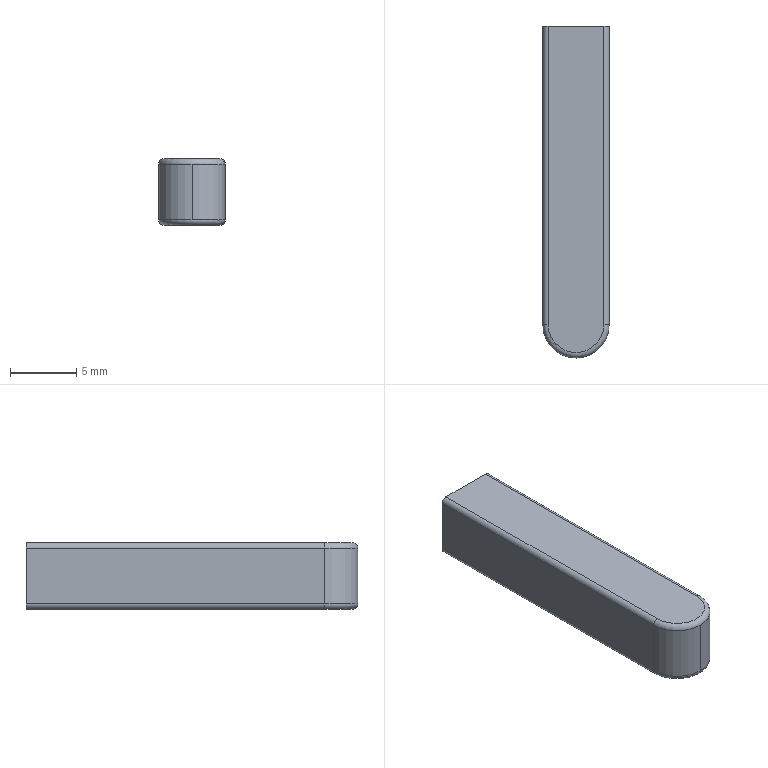Component | SolidWorks | GB_T1096-1979PlainParallelKeyC-type5_25-1 | 1 solid | 13 faces | box 5 x 25 x 5 mm | volume 608 mm3 | cylinder 6 | plane 5 | torus 2 | commonest cylinder face diameters 0.8 x4 5 x2
build123d program:
from build123d import *

# Parameters (mm, degrees)
BASE_EXTRUDE_DEPTH = 5
FILLET1_R          = 0.4


with BuildPart() as part:
    # Sketch1 → Base-Extrude (new body)
    with BuildSketch(Plane.XY):
        with BuildLine():
            Line((-9, 2.5), (13.5, 2.5))
            Line((13.5, 2.5), (13.5, -2.5))
            Line((13.5, -2.5), (-9, -2.5))
            ThreePointArc((-9, -2.5), (-11.5, 0), (-9, 2.5))
        make_face()
    extrude(amount=BASE_EXTRUDE_DEPTH)

    # Fillet1
    fillet1_edges = [part.edges().sort_by_distance(p)[0] for p in [
        (-11.5, 0, 5),
        (2.25, -2.5, 5),
        (2.25, -2.5, 0),
        (-11.5, 0, 0),
        (2.25, 2.5, 0),
        (2.25, 2.5, 5),
    ]]
    fillet(fillet1_edges, radius=FILLET1_R)


solid = part.part

# Placed as in the assembly
solid = solid.moved(Location((-96.534, 123.266, -174.507), (0, 0, 90)))
STEP:
#1=CARTESIAN_POINT('',(-3.702,4.499,-6.689));
#2=VERTEX_POINT('',#1);
#3=CARTESIAN_POINT('',(-3.801,4.4,-6.689));
#4=VERTEX_POINT('',#3);
#5=CARTESIAN_POINT('',(-3.801,4.499,-6.689));
#6=DIRECTION('',(-0.,0.,-1.));
#7=DIRECTION('',(0.,1.,0.));
#8=AXIS2_PLACEMENT_3D('',#5,#6,#7);
#9=CIRCLE('',#8,0.09843);
#10=EDGE_CURVE('',#2,#4,#9,.T.);
#11=ORIENTED_EDGE('',*,*,#10,.T.);
#12=CARTESIAN_POINT('',(-3.801,4.4,-6.855));
#13=VERTEX_POINT('',#12);
#14=CARTESIAN_POINT('',(-3.801,4.4,-6.674));
#15=DIRECTION('',(-0.,0.,-1.));
#16=VECTOR('',#15,39.37);
#17=LINE('',#14,#16);
#18=EDGE_CURVE('',#4,#13,#17,.T.);
#19=ORIENTED_EDGE('',*,*,#18,.T.);
#20=CARTESIAN_POINT('',(-3.702,4.499,-6.855));
#21=VERTEX_POINT('',#20);
#22=CARTESIAN_POINT('',(-3.801,4.499,-6.855));
#23=DIRECTION('',(0.,-0.,1.));
#24=DIRECTION('',(0.,1.,0.));
#25=AXIS2_PLACEMENT_3D('',#22,#23,#24);
#26=CIRCLE('',#25,0.09843);
#27=EDGE_CURVE('',#13,#21,#26,.T.);
#28=ORIENTED_EDGE('',*,*,#27,.T.);
#29=CARTESIAN_POINT('',(-3.702,4.499,-6.674));
#30=DIRECTION('',(-0.,0.,-1.));
#31=VECTOR('',#30,39.37);
#32=LINE('',#29,#31);
#33=EDGE_CURVE('',#2,#21,#32,.T.);
#34=ORIENTED_EDGE('',*,*,#33,.F.);
#35=EDGE_LOOP('',(#11,#19,#28,#34));
#36=FACE_OUTER_BOUND('',#35,.T.);
#37=CARTESIAN_POINT('',(-3.801,4.499,-6.674));
#38=DIRECTION('',(-0.,0.,-1.));
#39=DIRECTION('',(0.,-1.,0.));
#40=AXIS2_PLACEMENT_3D('',#37,#38,#39);
#41=CYLINDRICAL_SURFACE('',#40,0.09843);
#42=ADVANCED_FACE('',(#36),#41,.T.);
#43=CARTESIAN_POINT('',(-3.718,5.384,-6.674));
#44=VERTEX_POINT('',#43);
#45=CARTESIAN_POINT('',(-3.883,5.384,-6.674));
#46=VERTEX_POINT('',#45);
#47=CARTESIAN_POINT('',(-3.899,5.384,-6.674));
#48=DIRECTION('',(-1.,0.,0.));
#49=VECTOR('',#48,39.37);
#50=LINE('',#47,#49);
#51=EDGE_CURVE('',#44,#46,#50,.T.);
#52=ORIENTED_EDGE('',*,*,#51,.F.);
#53=CARTESIAN_POINT('',(-3.702,5.384,-6.689));
#54=VERTEX_POINT('',#53);
#55=CARTESIAN_POINT('',(-3.718,5.384,-6.689));
#56=DIRECTION('',(0.,1.,0.));
#57=DIRECTION('',(0.,0.,1.));
#58=AXIS2_PLACEMENT_3D('',#55,#56,#57);
#59=CIRCLE('',#58,0.01575);
#60=EDGE_CURVE('',#44,#54,#59,.T.);
#61=ORIENTED_EDGE('',*,*,#60,.T.);
#62=CARTESIAN_POINT('',(-3.702,5.384,-6.855));
#63=VERTEX_POINT('',#62);
#64=CARTESIAN_POINT('',(-3.702,5.384,-6.674));
#65=DIRECTION('',(-0.,0.,-1.));
#66=VECTOR('',#65,39.37);
#67=LINE('',#64,#66);
#68=EDGE_CURVE('',#54,#63,#67,.T.);
#69=ORIENTED_EDGE('',*,*,#68,.T.);
#70=CARTESIAN_POINT('',(-3.718,5.384,-6.87));
#71=VERTEX_POINT('',#70);
#72=CARTESIAN_POINT('',(-3.718,5.384,-6.855));
#73=DIRECTION('',(0.,1.,0.));
#74=DIRECTION('',(0.,0.,1.));
#75=AXIS2_PLACEMENT_3D('',#72,#73,#74);
#76=CIRCLE('',#75,0.01575);
#77=EDGE_CURVE('',#63,#71,#76,.T.);
#78=ORIENTED_EDGE('',*,*,#77,.T.);
#79=CARTESIAN_POINT('',(-3.883,5.384,-6.87));
#80=VERTEX_POINT('',#79);
#81=CARTESIAN_POINT('',(-3.899,5.384,-6.87));
#82=DIRECTION('',(-1.,0.,0.));
#83=VECTOR('',#82,39.37);
#84=LINE('',#81,#83);
#85=EDGE_CURVE('',#71,#80,#84,.T.);
#86=ORIENTED_EDGE('',*,*,#85,.T.);
#87=CARTESIAN_POINT('',(-3.899,5.384,-6.855));
#88=VERTEX_POINT('',#87);
#89=CARTESIAN_POINT('',(-3.883,5.384,-6.855));
#90=DIRECTION('',(0.,1.,0.));
#91=DIRECTION('',(0.,0.,1.));
#92=AXIS2_PLACEMENT_3D('',#89,#90,#91);
#93=CIRCLE('',#92,0.01575);
#94=EDGE_CURVE('',#80,#88,#93,.T.);
#95=ORIENTED_EDGE('',*,*,#94,.T.);
#96=CARTESIAN_POINT('',(-3.899,5.384,-6.689));
#97=VERTEX_POINT('',#96);
#98=CARTESIAN_POINT('',(-3.899,5.384,-6.674));
#99=DIRECTION('',(-0.,0.,-1.));
#100=VECTOR('',#99,39.37);
#101=LINE('',#98,#100);
#102=EDGE_CURVE('',#97,#88,#101,.T.);
#103=ORIENTED_EDGE('',*,*,#102,.F.);
#104=CARTESIAN_POINT('',(-3.883,5.384,-6.689));
#105=DIRECTION('',(0.,1.,0.));
#106=DIRECTION('',(0.,0.,1.));
#107=AXIS2_PLACEMENT_3D('',#104,#105,#106);
#108=CIRCLE('',#107,0.01575);
#109=EDGE_CURVE('',#97,#46,#108,.T.);
#110=ORIENTED_EDGE('',*,*,#109,.T.);
#111=EDGE_LOOP('',(#52,#61,#69,#78,#86,#95,#103,#110));
#112=FACE_OUTER_BOUND('',#111,.T.);
#113=CARTESIAN_POINT('',(-3.899,5.384,-6.674));
#114=DIRECTION('',(-0.,-1.,-0.));
#115=DIRECTION('',(0.,-0.,1.));
#116=AXIS2_PLACEMENT_3D('',#113,#114,#115);
#117=PLANE('',#116);
#118=ADVANCED_FACE('',(#112),#117,.F.);
#119=CARTESIAN_POINT('',(-3.899,4.499,-6.689));
#120=VERTEX_POINT('',#119);
#121=CARTESIAN_POINT('',(-3.899,4.499,-6.855));
#122=VERTEX_POINT('',#121);
#123=CARTESIAN_POINT('',(-3.899,4.499,-6.674));
#124=DIRECTION('',(-0.,0.,-1.));
#125=VECTOR('',#124,39.37);
#126=LINE('',#123,#125);
#127=EDGE_CURVE('',#120,#122,#126,.T.);
#128=ORIENTED_EDGE('',*,*,#127,.F.);
#129=CARTESIAN_POINT('',(-3.899,5.384,-6.689));
#130=DIRECTION('',(0.,1.,0.));
#131=VECTOR('',#130,39.37);
#132=LINE('',#129,#131);
#133=EDGE_CURVE('',#120,#97,#132,.T.);
#134=ORIENTED_EDGE('',*,*,#133,.T.);
#135=ORIENTED_EDGE('',*,*,#102,.T.);
#136=CARTESIAN_POINT('',(-3.899,4.499,-6.855));
#137=DIRECTION('',(-0.,-1.,-0.));
#138=VECTOR('',#137,39.37);
#139=LINE('',#136,#138);
#140=EDGE_CURVE('',#88,#122,#139,.T.);
#141=ORIENTED_EDGE('',*,*,#140,.T.);
#142=EDGE_LOOP('',(#128,#134,#135,#141));
#143=FACE_OUTER_BOUND('',#142,.T.);
#144=CARTESIAN_POINT('',(-3.899,4.499,-6.674));
#145=DIRECTION('',(1.,0.,-0.));
#146=DIRECTION('',(-0.,0.,-1.));
#147=AXIS2_PLACEMENT_3D('',#144,#145,#146);
#148=PLANE('',#147);
#149=ADVANCED_FACE('',(#143),#148,.F.);
#150=ORIENTED_EDGE('',*,*,#18,.F.);
#151=CARTESIAN_POINT('',(-3.801,4.499,-6.689));
#152=DIRECTION('',(-0.,0.,-1.));
#153=DIRECTION('',(0.,1.,0.));
#154=AXIS2_PLACEMENT_3D('',#151,#152,#153);
#155=CIRCLE('',#154,0.09843);
#156=EDGE_CURVE('',#4,#120,#155,.T.);
#157=ORIENTED_EDGE('',*,*,#156,.T.);
#158=ORIENTED_EDGE('',*,*,#127,.T.);
#159=CARTESIAN_POINT('',(-3.801,4.499,-6.855));
#160=DIRECTION('',(0.,-0.,1.));
#161=DIRECTION('',(0.,1.,0.));
#162=AXIS2_PLACEMENT_3D('',#159,#160,#161);
#163=CIRCLE('',#162,0.09843);
#164=EDGE_CURVE('',#122,#13,#163,.T.);
#165=ORIENTED_EDGE('',*,*,#164,.T.);
#166=EDGE_LOOP('',(#150,#157,#158,#165));
#167=FACE_OUTER_BOUND('',#166,.T.);
#168=CARTESIAN_POINT('',(-3.801,4.499,-6.674));
#169=DIRECTION('',(-0.,0.,-1.));
#170=DIRECTION('',(0.,-1.,0.));
#171=AXIS2_PLACEMENT_3D('',#168,#169,#170);
#172=CYLINDRICAL_SURFACE('',#171,0.09843);
#173=ADVANCED_FACE('',(#167),#172,.T.);
#174=ORIENTED_EDGE('',*,*,#68,.F.);
#175=CARTESIAN_POINT('',(-3.702,4.499,-6.689));
#176=DIRECTION('',(-0.,-1.,-0.));
#177=VECTOR('',#176,39.37);
#178=LINE('',#175,#177);
#179=EDGE_CURVE('',#54,#2,#178,.T.);
#180=ORIENTED_EDGE('',*,*,#179,.T.);
#181=ORIENTED_EDGE('',*,*,#33,.T.);
#182=CARTESIAN_POINT('',(-3.702,4.499,-6.855));
#183=DIRECTION('',(0.,1.,0.));
#184=VECTOR('',#183,39.37);
#185=LINE('',#182,#184);
#186=EDGE_CURVE('',#21,#63,#185,.T.);
#187=ORIENTED_EDGE('',*,*,#186,.T.);
#188=EDGE_LOOP('',(#174,#180,#181,#187));
#189=FACE_OUTER_BOUND('',#188,.T.);
#190=CARTESIAN_POINT('',(-3.702,4.499,-6.674));
#191=DIRECTION('',(-1.,0.,0.));
#192=DIRECTION('',(0.,-0.,1.));
#193=AXIS2_PLACEMENT_3D('',#190,#191,#192);
#194=PLANE('',#193);
#195=ADVANCED_FACE('',(#189),#194,.F.);
#196=CARTESIAN_POINT('',(-3.883,4.499,-6.674));
#197=VERTEX_POINT('',#196);
#198=CARTESIAN_POINT('',(-3.718,4.499,-6.674));
#199=VERTEX_POINT('',#198);
#200=CARTESIAN_POINT('',(-3.801,4.499,-6.674));
#201=DIRECTION('',(0.,-0.,1.));
#202=DIRECTION('',(0.,1.,0.));
#203=AXIS2_PLACEMENT_3D('',#200,#201,#202);
#204=CIRCLE('',#203,0.08268);
#205=EDGE_CURVE('',#197,#199,#204,.T.);
#206=ORIENTED_EDGE('',*,*,#205,.T.);
#207=CARTESIAN_POINT('',(-3.718,5.384,-6.674));
#208=DIRECTION('',(0.,1.,0.));
#209=VECTOR('',#208,39.37);
#210=LINE('',#207,#209);
#211=EDGE_CURVE('',#199,#44,#210,.T.);
#212=ORIENTED_EDGE('',*,*,#211,.T.);
#213=ORIENTED_EDGE('',*,*,#51,.T.);
#214=CARTESIAN_POINT('',(-3.883,4.499,-6.674));
#215=DIRECTION('',(-0.,-1.,-0.));
#216=VECTOR('',#215,39.37);
#217=LINE('',#214,#216);
#218=EDGE_CURVE('',#46,#197,#217,.T.);
#219=ORIENTED_EDGE('',*,*,#218,.T.);
#220=EDGE_LOOP('',(#206,#212,#213,#219));
#221=FACE_OUTER_BOUND('',#220,.T.);
#222=CARTESIAN_POINT('',(-3.801,4.499,-6.674));
#223=DIRECTION('',(0.,-0.,1.));
#224=DIRECTION('',(0.,1.,0.));
#225=AXIS2_PLACEMENT_3D('',#222,#223,#224);
#226=PLANE('',#225);
#227=ADVANCED_FACE('',(#221),#226,.T.);
#228=CARTESIAN_POINT('',(-3.718,4.499,-6.87));
#229=VERTEX_POINT('',#228);
#230=CARTESIAN_POINT('',(-3.883,4.499,-6.87));
#231=VERTEX_POINT('',#230);
#232=CARTESIAN_POINT('',(-3.801,4.499,-6.87));
#233=DIRECTION('',(-0.,0.,-1.));
#234=DIRECTION('',(0.,1.,0.));
#235=AXIS2_PLACEMENT_3D('',#232,#233,#234);
#236=CIRCLE('',#235,0.08268);
#237=EDGE_CURVE('',#229,#231,#236,.T.);
#238=ORIENTED_EDGE('',*,*,#237,.T.);
#239=CARTESIAN_POINT('',(-3.883,4.499,-6.87));
#240=DIRECTION('',(0.,1.,0.));
#241=VECTOR('',#240,39.37);
#242=LINE('',#239,#241);
#243=EDGE_CURVE('',#231,#80,#242,.T.);
#244=ORIENTED_EDGE('',*,*,#243,.T.);
#245=ORIENTED_EDGE('',*,*,#85,.F.);
#246=CARTESIAN_POINT('',(-3.718,4.499,-6.87));
#247=DIRECTION('',(-0.,-1.,-0.));
#248=VECTOR('',#247,39.37);
#249=LINE('',#246,#248);
#250=EDGE_CURVE('',#71,#229,#249,.T.);
#251=ORIENTED_EDGE('',*,*,#250,.T.);
#252=EDGE_LOOP('',(#238,#244,#245,#251));
#253=FACE_OUTER_BOUND('',#252,.T.);
#254=CARTESIAN_POINT('',(-3.801,4.499,-6.87));
#255=DIRECTION('',(0.,-0.,1.));
#256=DIRECTION('',(0.,1.,0.));
#257=AXIS2_PLACEMENT_3D('',#254,#255,#256);
#258=PLANE('',#257);
#259=ADVANCED_FACE('',(#253),#258,.F.);
#260=ORIENTED_EDGE('',*,*,#109,.F.);
#261=ORIENTED_EDGE('',*,*,#133,.F.);
#262=CARTESIAN_POINT('',(-3.883,4.499,-6.689));
#263=DIRECTION('',(-0.,-1.,-0.));
#264=DIRECTION('',(0.,0.,1.));
#265=AXIS2_PLACEMENT_3D('',#262,#263,#264);
#266=CIRCLE('',#265,0.01575);
#267=EDGE_CURVE('',#197,#120,#266,.T.);
#268=ORIENTED_EDGE('',*,*,#267,.F.);
#269=ORIENTED_EDGE('',*,*,#218,.F.);
#270=EDGE_LOOP('',(#260,#261,#268,#269));
#271=FACE_OUTER_BOUND('',#270,.T.);
#272=CARTESIAN_POINT('',(-3.883,4.499,-6.689));
#273=DIRECTION('',(0.,1.,0.));
#274=DIRECTION('',(0.,0.,-1.));
#275=AXIS2_PLACEMENT_3D('',#272,#273,#274);
#276=CYLINDRICAL_SURFACE('',#275,0.01575);
#277=ADVANCED_FACE('',(#271),#276,.T.);
#278=ORIENTED_EDGE('',*,*,#267,.T.);
#279=ORIENTED_EDGE('',*,*,#156,.F.);
#280=ORIENTED_EDGE('',*,*,#10,.F.);
#281=CARTESIAN_POINT('',(-3.718,4.499,-6.689));
#282=DIRECTION('',(0.,1.,0.));
#283=DIRECTION('',(0.,0.,-1.));
#284=AXIS2_PLACEMENT_3D('',#281,#282,#283);
#285=CIRCLE('',#284,0.01575);
#286=EDGE_CURVE('',#199,#2,#285,.T.);
#287=ORIENTED_EDGE('',*,*,#286,.F.);
#288=ORIENTED_EDGE('',*,*,#205,.F.);
#289=EDGE_LOOP('',(#278,#279,#280,#287,#288));
#290=FACE_OUTER_BOUND('',#289,.T.);
#291=CARTESIAN_POINT('',(-3.801,4.499,-6.689));
#292=DIRECTION('',(0.,-0.,1.));
#293=DIRECTION('',(0.,1.,0.));
#294=AXIS2_PLACEMENT_3D('',#291,#292,#293);
#295=TOROIDAL_SURFACE('',#294,0.08268,0.01575);
#296=ADVANCED_FACE('',(#290),#295,.T.);
#297=ORIENTED_EDGE('',*,*,#286,.T.);
#298=ORIENTED_EDGE('',*,*,#179,.F.);
#299=ORIENTED_EDGE('',*,*,#60,.F.);
#300=ORIENTED_EDGE('',*,*,#211,.F.);
#301=EDGE_LOOP('',(#297,#298,#299,#300));
#302=FACE_OUTER_BOUND('',#301,.T.);
#303=CARTESIAN_POINT('',(-3.718,4.499,-6.689));
#304=DIRECTION('',(-0.,-1.,-0.));
#305=DIRECTION('',(0.,0.,1.));
#306=AXIS2_PLACEMENT_3D('',#303,#304,#305);
#307=CYLINDRICAL_SURFACE('',#306,0.01575);
#308=ADVANCED_FACE('',(#302),#307,.T.);
#309=ORIENTED_EDGE('',*,*,#77,.F.);
#310=ORIENTED_EDGE('',*,*,#186,.F.);
#311=CARTESIAN_POINT('',(-3.718,4.499,-6.855));
#312=DIRECTION('',(-0.,-1.,-0.));
#313=DIRECTION('',(0.,0.,1.));
#314=AXIS2_PLACEMENT_3D('',#311,#312,#313);
#315=CIRCLE('',#314,0.01575);
#316=EDGE_CURVE('',#229,#21,#315,.T.);
#317=ORIENTED_EDGE('',*,*,#316,.F.);
#318=ORIENTED_EDGE('',*,*,#250,.F.);
#319=EDGE_LOOP('',(#309,#310,#317,#318));
#320=FACE_OUTER_BOUND('',#319,.T.);
#321=CARTESIAN_POINT('',(-3.718,4.499,-6.855));
#322=DIRECTION('',(0.,1.,0.));
#323=DIRECTION('',(0.,0.,-1.));
#324=AXIS2_PLACEMENT_3D('',#321,#322,#323);
#325=CYLINDRICAL_SURFACE('',#324,0.01575);
#326=ADVANCED_FACE('',(#320),#325,.T.);
#327=ORIENTED_EDGE('',*,*,#316,.T.);
#328=ORIENTED_EDGE('',*,*,#27,.F.);
#329=ORIENTED_EDGE('',*,*,#164,.F.);
#330=CARTESIAN_POINT('',(-3.883,4.499,-6.855));
#331=DIRECTION('',(0.,1.,0.));
#332=DIRECTION('',(0.,0.,-1.));
#333=AXIS2_PLACEMENT_3D('',#330,#331,#332);
#334=CIRCLE('',#333,0.01575);
#335=EDGE_CURVE('',#231,#122,#334,.T.);
#336=ORIENTED_EDGE('',*,*,#335,.F.);
#337=ORIENTED_EDGE('',*,*,#237,.F.);
#338=EDGE_LOOP('',(#327,#328,#329,#336,#337));
#339=FACE_OUTER_BOUND('',#338,.T.);
#340=CARTESIAN_POINT('',(-3.801,4.499,-6.855));
#341=DIRECTION('',(0.,-0.,1.));
#342=DIRECTION('',(0.,1.,0.));
#343=AXIS2_PLACEMENT_3D('',#340,#341,#342);
#344=TOROIDAL_SURFACE('',#343,0.08268,0.01575);
#345=ADVANCED_FACE('',(#339),#344,.T.);
#346=ORIENTED_EDGE('',*,*,#94,.F.);
#347=ORIENTED_EDGE('',*,*,#243,.F.);
#348=ORIENTED_EDGE('',*,*,#335,.T.);
#349=ORIENTED_EDGE('',*,*,#140,.F.);
#350=EDGE_LOOP('',(#346,#347,#348,#349));
#351=FACE_OUTER_BOUND('',#350,.T.);
#352=CARTESIAN_POINT('',(-3.883,4.499,-6.855));
#353=DIRECTION('',(-0.,-1.,-0.));
#354=DIRECTION('',(0.,0.,1.));
#355=AXIS2_PLACEMENT_3D('',#352,#353,#354);
#356=CYLINDRICAL_SURFACE('',#355,0.01575);
#357=ADVANCED_FACE('',(#351),#356,.T.);
#358=CLOSED_SHELL('',(#42,#118,#149,#173,#195,#227,#259,#277,#296,#308,#326,#345,#357));
#359=MANIFOLD_SOLID_BREP('',#358);
#360=CARTESIAN_POINT('',(0.,0.,0.));
#361=DIRECTION('',(0.,0.,1.));
#362=DIRECTION('',(1.,0.,0.));
#363=AXIS2_PLACEMENT_3D('',#360,#361,#362);
#364=(LENGTH_UNIT()NAMED_UNIT(*)SI_UNIT($,.METRE.));
#365=LENGTH_MEASURE_WITH_UNIT(LENGTH_MEASURE(0.0254),#364);
#366=DIMENSIONAL_EXPONENTS(1.,0.,0.,0.,0.,0.,0.);
#367=(CONVERSION_BASED_UNIT('',#365)LENGTH_UNIT()NAMED_UNIT(#366));
#368=UNCERTAINTY_MEASURE_WITH_UNIT(LENGTH_MEASURE(0.00001),#367,'','');
#369=(NAMED_UNIT(*)PLANE_ANGLE_UNIT()SI_UNIT($,.RADIAN.));
#370=(NAMED_UNIT(*)SI_UNIT($,.STERADIAN.)SOLID_ANGLE_UNIT());
#371=(GEOMETRIC_REPRESENTATION_CONTEXT(3)GLOBAL_UNCERTAINTY_ASSIGNED_CONTEXT((#368))GLOBAL_UNIT_ASSIGNED_CONTEXT((#367,#369,#370))REPRESENTATION_CONTEXT('',''));
#372=ADVANCED_BREP_SHAPE_REPRESENTATION('',(#359,#363),#371);
#373=COLOUR_RGB('',0.7922,0.8196,0.9333);
#374=FILL_AREA_STYLE_COLOUR('',#373);
#375=FILL_AREA_STYLE('',(#374));
#376=SURFACE_STYLE_FILL_AREA(#375);
#377=SURFACE_SIDE_STYLE('',(#376));
#378=SURFACE_STYLE_USAGE(.BOTH.,#377);
#379=PRESENTATION_STYLE_ASSIGNMENT((#378));
#380=STYLED_ITEM('',(#379),#359);
#381=(LENGTH_UNIT()NAMED_UNIT(*)SI_UNIT($,.METRE.));
#382=LENGTH_MEASURE_WITH_UNIT(LENGTH_MEASURE(0.0254),#381);
#383=DIMENSIONAL_EXPONENTS(1.,0.,0.,0.,0.,0.,0.);
#384=(CONVERSION_BASED_UNIT('',#382)LENGTH_UNIT()NAMED_UNIT(#383));
#385=UNCERTAINTY_MEASURE_WITH_UNIT(LENGTH_MEASURE(0.00001),#384,'','');
#386=(NAMED_UNIT(*)PLANE_ANGLE_UNIT()SI_UNIT($,.RADIAN.));
#387=(NAMED_UNIT(*)SI_UNIT($,.STERADIAN.)SOLID_ANGLE_UNIT());
#388=(GEOMETRIC_REPRESENTATION_CONTEXT(3)GLOBAL_UNCERTAINTY_ASSIGNED_CONTEXT((#385))GLOBAL_UNIT_ASSIGNED_CONTEXT((#384,#386,#387))REPRESENTATION_CONTEXT('',''));
#389=MECHANICAL_DESIGN_GEOMETRIC_PRESENTATION_REPRESENTATION('',(#380),#388);
#390=PRESENTATION_LAYER_ASSIGNMENT('','',(#380));